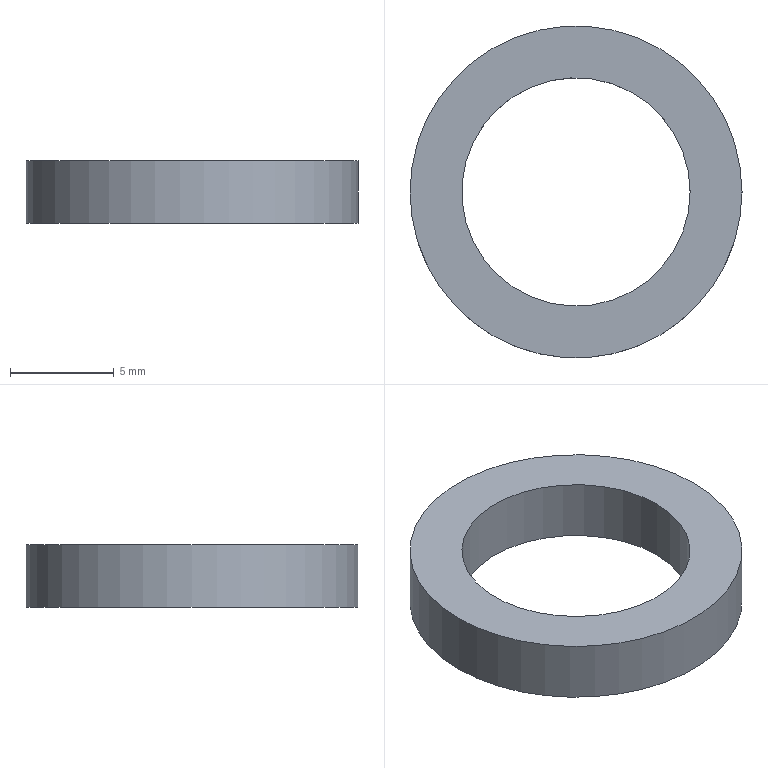Component | NX | M10_WASHER_3 | 1 solid | 4 faces | box 16 x 16 x 3 mm | volume 318 mm3 | cylinder 2 | plane 2 | commonest cylinder face diameters 16 x1 11 x1
STEP:
#1=CARTESIAN_POINT('',(0.,0.,0.));
#2=DIRECTION('',(0.,0.,1.));
#3=DIRECTION('',(1.,0.,0.));
#4=AXIS2_PLACEMENT_3D('',#1,#2,#3);
#5=CARTESIAN_POINT('',(-144.594,113.985,13.));
#6=VERTEX_POINT('',#5);
#7=CARTESIAN_POINT('',(-152.594,113.985,13.));
#8=DIRECTION('',(0.,0.,1.));
#9=DIRECTION('',(1.,0.,0.));
#10=AXIS2_PLACEMENT_3D('',#7,#8,#9);
#11=CIRCLE('',#10,8.);
#12=CARTESIAN_POINT('',(-152.594,113.985,13.));
#13=DIRECTION('',(0.,0.,-1.));
#14=DIRECTION('',(-1.,0.,0.));
#15=AXIS2_PLACEMENT_3D('',#12,#13,#14);
#16=CYLINDRICAL_SURFACE('',#15,8.);
#17=CARTESIAN_POINT('',(9.425,0.));
#18=DIRECTION('',(-1.,0.));
#19=VECTOR('',#18,1.);
#20=LINE('',#17,#19);
#21=(GEOMETRIC_REPRESENTATION_CONTEXT(2)PARAMETRIC_REPRESENTATION_CONTEXT()REPRESENTATION_CONTEXT('',''));
#22=DEFINITIONAL_REPRESENTATION('',(#20),#21);
#23=PCURVE('',#16,#22);
#24=CARTESIAN_POINT('',(-152.594,113.985,13.));
#25=DIRECTION('',(0.,0.,1.));
#26=DIRECTION('',(1.,0.,0.));
#27=AXIS2_PLACEMENT_3D('',#24,#25,#26);
#28=PLANE('',#27);
#29=CARTESIAN_POINT('',(0.,0.));
#30=DIRECTION('',(1.,0.));
#31=AXIS2_PLACEMENT_2D('',#29,#30);
#32=CIRCLE('',#31,8.);
#33=(GEOMETRIC_REPRESENTATION_CONTEXT(2)PARAMETRIC_REPRESENTATION_CONTEXT()REPRESENTATION_CONTEXT('',''));
#34=DEFINITIONAL_REPRESENTATION('',(#32),#33);
#35=PCURVE('',#28,#34);
#36=SURFACE_CURVE('',#11,(#23,#35),.PCURVE_S1.);
#37=EDGE_CURVE('',#6,#6,#36,.T.);
#38=ORIENTED_EDGE('',*,*,#37,.F.);
#39=CARTESIAN_POINT('',(-144.594,113.985,10.));
#40=VERTEX_POINT('',#39);
#41=CARTESIAN_POINT('',(-144.594,113.985,13.));
#42=CARTESIAN_POINT('',(-144.594,113.985,10.));
#43=B_SPLINE_CURVE_WITH_KNOTS('',1,(#41,#42),.UNSPECIFIED.,.F.,.F.,(2,2),(0.,3.),.PIECEWISE_BEZIER_KNOTS.);
#44=CARTESIAN_POINT('',(9.425,0.));
#45=DIRECTION('',(0.,1.));
#46=VECTOR('',#45,1.);
#47=LINE('',#44,#46);
#48=(GEOMETRIC_REPRESENTATION_CONTEXT(2)PARAMETRIC_REPRESENTATION_CONTEXT()REPRESENTATION_CONTEXT('',''));
#49=DEFINITIONAL_REPRESENTATION('',(#47),#48);
#50=PCURVE('',#16,#49);
#51=CARTESIAN_POINT('',(3.142,0.));
#52=DIRECTION('',(0.,1.));
#53=VECTOR('',#52,1.);
#54=LINE('',#51,#53);
#55=(GEOMETRIC_REPRESENTATION_CONTEXT(2)PARAMETRIC_REPRESENTATION_CONTEXT()REPRESENTATION_CONTEXT('',''));
#56=DEFINITIONAL_REPRESENTATION('',(#54),#55);
#57=PCURVE('',#16,#56);
#58=SEAM_CURVE('',#43,(#50,#57),.PCURVE_S1.);
#59=EDGE_CURVE('',#6,#40,#58,.T.);
#60=ORIENTED_EDGE('',*,*,#59,.T.);
#61=CARTESIAN_POINT('',(-152.594,113.985,10.));
#62=DIRECTION('',(0.,0.,1.));
#63=DIRECTION('',(1.,0.,0.));
#64=AXIS2_PLACEMENT_3D('',#61,#62,#63);
#65=CIRCLE('',#64,8.);
#66=CARTESIAN_POINT('',(9.425,3.));
#67=DIRECTION('',(-1.,0.));
#68=VECTOR('',#67,1.);
#69=LINE('',#66,#68);
#70=(GEOMETRIC_REPRESENTATION_CONTEXT(2)PARAMETRIC_REPRESENTATION_CONTEXT()REPRESENTATION_CONTEXT('',''));
#71=DEFINITIONAL_REPRESENTATION('',(#69),#70);
#72=PCURVE('',#16,#71);
#73=CARTESIAN_POINT('',(-152.594,113.985,10.));
#74=DIRECTION('',(0.,0.,1.));
#75=DIRECTION('',(1.,0.,0.));
#76=AXIS2_PLACEMENT_3D('',#73,#74,#75);
#77=PLANE('',#76);
#78=CARTESIAN_POINT('',(0.,0.));
#79=DIRECTION('',(1.,0.));
#80=AXIS2_PLACEMENT_2D('',#78,#79);
#81=CIRCLE('',#80,8.);
#82=(GEOMETRIC_REPRESENTATION_CONTEXT(2)PARAMETRIC_REPRESENTATION_CONTEXT()REPRESENTATION_CONTEXT('',''));
#83=DEFINITIONAL_REPRESENTATION('',(#81),#82);
#84=PCURVE('',#77,#83);
#85=SURFACE_CURVE('',#65,(#72,#84),.PCURVE_S1.);
#86=EDGE_CURVE('',#40,#40,#85,.T.);
#87=ORIENTED_EDGE('',*,*,#86,.T.);
#88=ORIENTED_EDGE('',*,*,#59,.F.);
#89=EDGE_LOOP('',(#38,#60,#87,#88));
#90=FACE_BOUND('',#89,.T.);
#91=ADVANCED_FACE('',(#90),#16,.T.);
#92=CARTESIAN_POINT('',(-147.094,113.985,13.));
#93=VERTEX_POINT('',#92);
#94=CARTESIAN_POINT('',(-152.594,113.985,13.));
#95=DIRECTION('',(0.,0.,1.));
#96=DIRECTION('',(1.,0.,0.));
#97=AXIS2_PLACEMENT_3D('',#94,#95,#96);
#98=CIRCLE('',#97,5.5);
#99=CARTESIAN_POINT('',(-152.594,113.985,13.));
#100=DIRECTION('',(0.,0.,-1.));
#101=DIRECTION('',(-1.,0.,0.));
#102=AXIS2_PLACEMENT_3D('',#99,#100,#101);
#103=CYLINDRICAL_SURFACE('',#102,5.5);
#104=CARTESIAN_POINT('',(9.425,0.));
#105=DIRECTION('',(-1.,0.));
#106=VECTOR('',#105,1.);
#107=LINE('',#104,#106);
#108=(GEOMETRIC_REPRESENTATION_CONTEXT(2)PARAMETRIC_REPRESENTATION_CONTEXT()REPRESENTATION_CONTEXT('',''));
#109=DEFINITIONAL_REPRESENTATION('',(#107),#108);
#110=PCURVE('',#103,#109);
#111=CARTESIAN_POINT('',(0.,0.));
#112=DIRECTION('',(1.,0.));
#113=AXIS2_PLACEMENT_2D('',#111,#112);
#114=CIRCLE('',#113,5.5);
#115=(GEOMETRIC_REPRESENTATION_CONTEXT(2)PARAMETRIC_REPRESENTATION_CONTEXT()REPRESENTATION_CONTEXT('',''));
#116=DEFINITIONAL_REPRESENTATION('',(#114),#115);
#117=PCURVE('',#28,#116);
#118=SURFACE_CURVE('',#98,(#110,#117),.PCURVE_S1.);
#119=EDGE_CURVE('',#93,#93,#118,.T.);
#120=ORIENTED_EDGE('',*,*,#119,.F.);
#121=CARTESIAN_POINT('',(-147.094,113.985,10.));
#122=VERTEX_POINT('',#121);
#123=CARTESIAN_POINT('',(-147.094,113.985,13.));
#124=CARTESIAN_POINT('',(-147.094,113.985,10.));
#125=B_SPLINE_CURVE_WITH_KNOTS('',1,(#123,#124),.UNSPECIFIED.,.F.,.F.,(2,2),(0.,3.),.PIECEWISE_BEZIER_KNOTS.);
#126=CARTESIAN_POINT('',(9.425,0.));
#127=DIRECTION('',(0.,1.));
#128=VECTOR('',#127,1.);
#129=LINE('',#126,#128);
#130=(GEOMETRIC_REPRESENTATION_CONTEXT(2)PARAMETRIC_REPRESENTATION_CONTEXT()REPRESENTATION_CONTEXT('',''));
#131=DEFINITIONAL_REPRESENTATION('',(#129),#130);
#132=PCURVE('',#103,#131);
#133=CARTESIAN_POINT('',(3.142,0.));
#134=DIRECTION('',(0.,1.));
#135=VECTOR('',#134,1.);
#136=LINE('',#133,#135);
#137=(GEOMETRIC_REPRESENTATION_CONTEXT(2)PARAMETRIC_REPRESENTATION_CONTEXT()REPRESENTATION_CONTEXT('',''));
#138=DEFINITIONAL_REPRESENTATION('',(#136),#137);
#139=PCURVE('',#103,#138);
#140=SEAM_CURVE('',#125,(#132,#139),.PCURVE_S1.);
#141=EDGE_CURVE('',#93,#122,#140,.T.);
#142=ORIENTED_EDGE('',*,*,#141,.T.);
#143=CARTESIAN_POINT('',(-152.594,113.985,10.));
#144=DIRECTION('',(0.,0.,1.));
#145=DIRECTION('',(1.,0.,0.));
#146=AXIS2_PLACEMENT_3D('',#143,#144,#145);
#147=CIRCLE('',#146,5.5);
#148=CARTESIAN_POINT('',(9.425,3.));
#149=DIRECTION('',(-1.,0.));
#150=VECTOR('',#149,1.);
#151=LINE('',#148,#150);
#152=(GEOMETRIC_REPRESENTATION_CONTEXT(2)PARAMETRIC_REPRESENTATION_CONTEXT()REPRESENTATION_CONTEXT('',''));
#153=DEFINITIONAL_REPRESENTATION('',(#151),#152);
#154=PCURVE('',#103,#153);
#155=CARTESIAN_POINT('',(0.,0.));
#156=DIRECTION('',(1.,0.));
#157=AXIS2_PLACEMENT_2D('',#155,#156);
#158=CIRCLE('',#157,5.5);
#159=(GEOMETRIC_REPRESENTATION_CONTEXT(2)PARAMETRIC_REPRESENTATION_CONTEXT()REPRESENTATION_CONTEXT('',''));
#160=DEFINITIONAL_REPRESENTATION('',(#158),#159);
#161=PCURVE('',#77,#160);
#162=SURFACE_CURVE('',#147,(#154,#161),.PCURVE_S1.);
#163=EDGE_CURVE('',#122,#122,#162,.T.);
#164=ORIENTED_EDGE('',*,*,#163,.T.);
#165=ORIENTED_EDGE('',*,*,#141,.F.);
#166=EDGE_LOOP('',(#120,#142,#164,#165));
#167=FACE_BOUND('',#166,.F.);
#168=ADVANCED_FACE('',(#167),#103,.F.);
#169=ORIENTED_EDGE('',*,*,#37,.T.);
#170=EDGE_LOOP('',(#169));
#171=FACE_BOUND('',#170,.T.);
#172=ORIENTED_EDGE('',*,*,#119,.F.);
#173=EDGE_LOOP('',(#172));
#174=FACE_BOUND('',#173,.T.);
#175=ADVANCED_FACE('',(#171,#174),#28,.T.);
#176=ORIENTED_EDGE('',*,*,#86,.F.);
#177=EDGE_LOOP('',(#176));
#178=FACE_BOUND('',#177,.T.);
#179=ORIENTED_EDGE('',*,*,#163,.T.);
#180=EDGE_LOOP('',(#179));
#181=FACE_BOUND('',#180,.T.);
#182=ADVANCED_FACE('',(#178,#181),#77,.F.);
#183=CLOSED_SHELL('',(#91,#168,#175,#182));
#184=MANIFOLD_SOLID_BREP('',#183);
#185=(LENGTH_UNIT()NAMED_UNIT(*)SI_UNIT(.MILLI.,.METRE.));
#186=UNCERTAINTY_MEASURE_WITH_UNIT(LENGTH_MEASURE(0.00001),#185,'','');
#187=(NAMED_UNIT(*)PLANE_ANGLE_UNIT()SI_UNIT($,.RADIAN.));
#188=(NAMED_UNIT(*)SI_UNIT($,.STERADIAN.)SOLID_ANGLE_UNIT());
#189=(GEOMETRIC_REPRESENTATION_CONTEXT(3)GLOBAL_UNCERTAINTY_ASSIGNED_CONTEXT((#186))GLOBAL_UNIT_ASSIGNED_CONTEXT((#185,#187,#188))REPRESENTATION_CONTEXT('',''));
#190=ADVANCED_BREP_SHAPE_REPRESENTATION('',(#4,#184),#189);